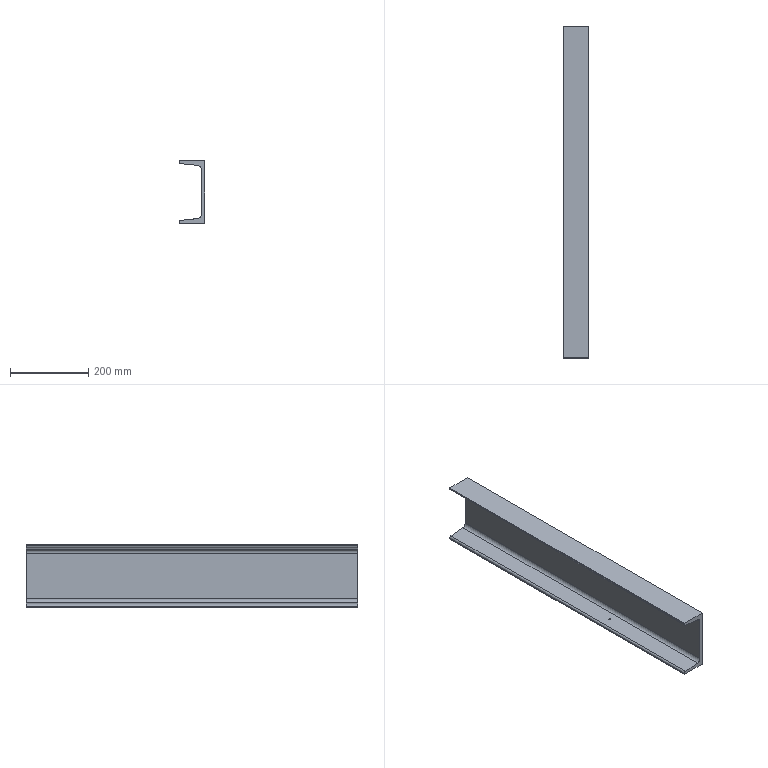Component | SolidWorks | NitrogenSupportChannelSteel65016a-331MachineTool-1 | 1 solid | 16 faces | box 65 x 850 x 160 mm | volume 2137904 mm3 | plane 10 | cylinder 6 | commonest cylinder face diameters 5 x2 20 x2 10 x2
STEP:
#1=COLOUR_RGB('',0.7922,0.8196,0.9333);
#2=FILL_AREA_STYLE_COLOUR('',#1);
#3=FILL_AREA_STYLE('',(#2));
#4=SURFACE_STYLE_FILL_AREA(#3);
#5=SURFACE_SIDE_STYLE('',(#4));
#6=SURFACE_STYLE_USAGE(.BOTH.,#5);
#7=PRESENTATION_STYLE_ASSIGNMENT((#6));
#8=CARTESIAN_POINT('',(1.747,6.759,23.228));
#9=VERTEX_POINT('',#8);
#10=CARTESIAN_POINT('',(1.945,6.759,23.228));
#11=VERTEX_POINT('',#10);
#12=CARTESIAN_POINT('',(1.747,6.759,23.228));
#13=CARTESIAN_POINT('',(1.747,6.956,23.228));
#14=CARTESIAN_POINT('',(1.945,6.956,23.228));
#15=CARTESIAN_POINT('',(1.945,6.759,23.228));
#16=(BOUNDED_CURVE()B_SPLINE_CURVE(3,(#12,#13,#14,#15),.UNSPECIFIED.,.F.,.T.)B_SPLINE_CURVE_WITH_KNOTS((4,4),(0.,3.142),.UNSPECIFIED.)CURVE()GEOMETRIC_REPRESENTATION_ITEM()RATIONAL_B_SPLINE_CURVE((1.,0.3333,0.3333,1.))REPRESENTATION_ITEM(''));
#17=EDGE_CURVE('',#9,#11,#16,.T.);
#18=ORIENTED_EDGE('',*,*,#17,.T.);
#19=CARTESIAN_POINT('',(1.905,6.759,23.632));
#20=VERTEX_POINT('',#19);
#21=CARTESIAN_POINT('',(1.905,6.759,23.632));
#22=DIRECTION('',(-0.0995,0.,0.995));
#23=VECTOR('',#22,39.37);
#24=LINE('',#21,#23);
#25=EDGE_CURVE('',#11,#20,#24,.T.);
#26=ORIENTED_EDGE('',*,*,#25,.T.);
#27=CARTESIAN_POINT('',(1.709,6.759,23.612));
#28=VERTEX_POINT('',#27);
#29=CARTESIAN_POINT('',(1.807,6.759,23.622));
#30=DIRECTION('',(-0.0995,0.,0.995));
#31=DIRECTION('',(-0.995,0.,-0.0995));
#32=AXIS2_PLACEMENT_3D('',#29,#30,#31);
#33=CIRCLE('',#32,0.09843);
#34=EDGE_CURVE('',#20,#28,#33,.T.);
#35=ORIENTED_EDGE('',*,*,#34,.T.);
#36=CARTESIAN_POINT('',(1.709,6.759,23.612));
#37=DIRECTION('',(-0.0995,0.,0.995));
#38=VECTOR('',#37,39.37);
#39=LINE('',#36,#38);
#40=EDGE_CURVE('',#9,#28,#39,.T.);
#41=ORIENTED_EDGE('',*,*,#40,.F.);
#42=EDGE_LOOP('',(#18,#26,#35,#41));
#43=FACE_OUTER_BOUND('',#42,.T.);
#44=CARTESIAN_POINT('',(1.807,6.759,23.622));
#45=DIRECTION('',(-0.0995,0.,0.995));
#46=DIRECTION('',(-0.995,0.,-0.0995));
#47=AXIS2_PLACEMENT_3D('',#44,#45,#46);
#48=CYLINDRICAL_SURFACE('',#47,0.09843);
#49=ADVANCED_FACE('',(#43),#48,.F.);
#50=CARTESIAN_POINT('',(2.567,28.482,23.698));
#51=VERTEX_POINT('',#50);
#52=CARTESIAN_POINT('',(2.922,28.482,24.09));
#53=VERTEX_POINT('',#52);
#54=CARTESIAN_POINT('',(2.528,28.482,24.09));
#55=DIRECTION('',(0.,-1.,-0.));
#56=DIRECTION('',(-1.,0.,0.));
#57=AXIS2_PLACEMENT_3D('',#54,#55,#56);
#58=CIRCLE('',#57,0.3937);
#59=EDGE_CURVE('',#51,#53,#58,.T.);
#60=ORIENTED_EDGE('',*,*,#59,.F.);
#61=CARTESIAN_POINT('',(2.567,-4.983,23.698));
#62=VERTEX_POINT('',#61);
#63=CARTESIAN_POINT('',(2.567,-4.983,23.698));
#64=DIRECTION('',(-0.,1.,0.));
#65=VECTOR('',#64,39.37);
#66=LINE('',#63,#65);
#67=EDGE_CURVE('',#62,#51,#66,.T.);
#68=ORIENTED_EDGE('',*,*,#67,.F.);
#69=CARTESIAN_POINT('',(2.922,-4.983,24.09));
#70=VERTEX_POINT('',#69);
#71=CARTESIAN_POINT('',(2.528,-4.983,24.09));
#72=DIRECTION('',(0.,-1.,-0.));
#73=DIRECTION('',(-1.,0.,0.));
#74=AXIS2_PLACEMENT_3D('',#71,#72,#73);
#75=CIRCLE('',#74,0.3937);
#76=EDGE_CURVE('',#62,#70,#75,.T.);
#77=ORIENTED_EDGE('',*,*,#76,.T.);
#78=CARTESIAN_POINT('',(2.922,-4.983,24.09));
#79=DIRECTION('',(-0.,1.,0.));
#80=VECTOR('',#79,39.37);
#81=LINE('',#78,#80);
#82=EDGE_CURVE('',#70,#53,#81,.T.);
#83=ORIENTED_EDGE('',*,*,#82,.T.);
#84=EDGE_LOOP('',(#60,#68,#77,#83));
#85=FACE_OUTER_BOUND('',#84,.T.);
#86=CARTESIAN_POINT('',(2.528,-4.983,24.09));
#87=DIRECTION('',(-0.,1.,0.));
#88=DIRECTION('',(1.,0.,0.));
#89=AXIS2_PLACEMENT_3D('',#86,#87,#88);
#90=CYLINDRICAL_SURFACE('',#89,0.3937);
#91=ADVANCED_FACE('',(#85),#90,.F.);
#92=CARTESIAN_POINT('',(1.807,6.759,23.622));
#93=DIRECTION('',(-0.0995,0.,0.995));
#94=DIRECTION('',(-0.995,0.,-0.0995));
#95=AXIS2_PLACEMENT_3D('',#92,#93,#94);
#96=CIRCLE('',#95,0.09843);
#97=EDGE_CURVE('',#28,#20,#96,.T.);
#98=ORIENTED_EDGE('',*,*,#97,.F.);
#99=ORIENTED_EDGE('',*,*,#34,.F.);
#100=EDGE_LOOP('',(#98,#99));
#101=FACE_BOUND('',#100,.T.);
#102=CARTESIAN_POINT('',(0.8749,28.482,23.529));
#103=VERTEX_POINT('',#102);
#104=CARTESIAN_POINT('',(0.8749,28.482,23.529));
#105=DIRECTION('',(0.995,-0.,0.0995));
#106=VECTOR('',#105,39.37);
#107=LINE('',#104,#106);
#108=EDGE_CURVE('',#103,#51,#107,.T.);
#109=ORIENTED_EDGE('',*,*,#108,.F.);
#110=CARTESIAN_POINT('',(0.8749,-4.983,23.529));
#111=VERTEX_POINT('',#110);
#112=CARTESIAN_POINT('',(0.8749,-4.983,23.529));
#113=DIRECTION('',(-0.,1.,0.));
#114=VECTOR('',#113,39.37);
#115=LINE('',#112,#114);
#116=EDGE_CURVE('',#111,#103,#115,.T.);
#117=ORIENTED_EDGE('',*,*,#116,.F.);
#118=CARTESIAN_POINT('',(0.8749,-4.983,23.529));
#119=DIRECTION('',(0.995,-0.,0.0995));
#120=VECTOR('',#119,39.37);
#121=LINE('',#118,#120);
#122=EDGE_CURVE('',#111,#62,#121,.T.);
#123=ORIENTED_EDGE('',*,*,#122,.T.);
#124=ORIENTED_EDGE('',*,*,#67,.T.);
#125=EDGE_LOOP('',(#109,#117,#123,#124));
#126=FACE_OUTER_BOUND('',#125,.T.);
#127=CARTESIAN_POINT('',(0.8749,-4.983,23.529));
#128=DIRECTION('',(-0.0995,0.,0.995));
#129=DIRECTION('',(-0.995,0.,-0.0995));
#130=AXIS2_PLACEMENT_3D('',#127,#128,#129);
#131=PLANE('',#130);
#132=ADVANCED_FACE('',(#101,#126),#131,.T.);
#133=CARTESIAN_POINT('',(0.6976,28.482,23.333));
#134=VERTEX_POINT('',#133);
#135=CARTESIAN_POINT('',(0.8945,28.482,23.333));
#136=DIRECTION('',(-0.,1.,0.));
#137=DIRECTION('',(1.,0.,0.));
#138=AXIS2_PLACEMENT_3D('',#135,#136,#137);
#139=CIRCLE('',#138,0.1969);
#140=EDGE_CURVE('',#134,#103,#139,.T.);
#141=ORIENTED_EDGE('',*,*,#140,.F.);
#142=CARTESIAN_POINT('',(0.6976,-4.983,23.333));
#143=VERTEX_POINT('',#142);
#144=CARTESIAN_POINT('',(0.6976,-4.983,23.333));
#145=DIRECTION('',(-0.,1.,0.));
#146=VECTOR('',#145,39.37);
#147=LINE('',#144,#146);
#148=EDGE_CURVE('',#143,#134,#147,.T.);
#149=ORIENTED_EDGE('',*,*,#148,.F.);
#150=CARTESIAN_POINT('',(0.8945,-4.983,23.333));
#151=DIRECTION('',(-0.,1.,0.));
#152=DIRECTION('',(1.,0.,0.));
#153=AXIS2_PLACEMENT_3D('',#150,#151,#152);
#154=CIRCLE('',#153,0.1969);
#155=EDGE_CURVE('',#143,#111,#154,.T.);
#156=ORIENTED_EDGE('',*,*,#155,.T.);
#157=ORIENTED_EDGE('',*,*,#116,.T.);
#158=EDGE_LOOP('',(#141,#149,#156,#157));
#159=FACE_OUTER_BOUND('',#158,.T.);
#160=CARTESIAN_POINT('',(0.8945,-4.983,23.333));
#161=DIRECTION('',(-0.,1.,0.));
#162=DIRECTION('',(1.,0.,0.));
#163=AXIS2_PLACEMENT_3D('',#160,#161,#162);
#164=CYLINDRICAL_SURFACE('',#163,0.1969);
#165=ADVANCED_FACE('',(#159),#164,.T.);
#166=CARTESIAN_POINT('',(0.6976,28.482,23.228));
#167=VERTEX_POINT('',#166);
#168=CARTESIAN_POINT('',(0.6976,28.482,23.228));
#169=DIRECTION('',(-0.,0.,1.));
#170=VECTOR('',#169,39.37);
#171=LINE('',#168,#170);
#172=EDGE_CURVE('',#167,#134,#171,.T.);
#173=ORIENTED_EDGE('',*,*,#172,.F.);
#174=CARTESIAN_POINT('',(0.6976,-4.983,23.228));
#175=VERTEX_POINT('',#174);
#176=CARTESIAN_POINT('',(0.6976,-4.983,23.228));
#177=DIRECTION('',(-0.,1.,0.));
#178=VECTOR('',#177,39.37);
#179=LINE('',#176,#178);
#180=EDGE_CURVE('',#175,#167,#179,.T.);
#181=ORIENTED_EDGE('',*,*,#180,.F.);
#182=CARTESIAN_POINT('',(0.6976,-4.983,23.228));
#183=DIRECTION('',(-0.,0.,1.));
#184=VECTOR('',#183,39.37);
#185=LINE('',#182,#184);
#186=EDGE_CURVE('',#175,#143,#185,.T.);
#187=ORIENTED_EDGE('',*,*,#186,.T.);
#188=ORIENTED_EDGE('',*,*,#148,.T.);
#189=EDGE_LOOP('',(#173,#181,#187,#188));
#190=FACE_OUTER_BOUND('',#189,.T.);
#191=CARTESIAN_POINT('',(0.6976,-4.983,23.228));
#192=DIRECTION('',(-1.,-0.,0.));
#193=DIRECTION('',(-0.,1.,0.));
#194=AXIS2_PLACEMENT_3D('',#191,#192,#193);
#195=PLANE('',#194);
#196=ADVANCED_FACE('',(#190),#195,.T.);
#197=ORIENTED_EDGE('',*,*,#17,.F.);
#198=CARTESIAN_POINT('',(1.945,6.759,23.228));
#199=CARTESIAN_POINT('',(1.945,6.563,23.228));
#200=CARTESIAN_POINT('',(1.747,6.563,23.228));
#201=CARTESIAN_POINT('',(1.747,6.759,23.228));
#202=(BOUNDED_CURVE()B_SPLINE_CURVE(3,(#198,#199,#200,#201),.UNSPECIFIED.,.F.,.T.)B_SPLINE_CURVE_WITH_KNOTS((4,4),(3.142,6.283),.UNSPECIFIED.)CURVE()GEOMETRIC_REPRESENTATION_ITEM()RATIONAL_B_SPLINE_CURVE((1.,0.3333,0.3333,1.))REPRESENTATION_ITEM(''));
#203=EDGE_CURVE('',#11,#9,#202,.T.);
#204=ORIENTED_EDGE('',*,*,#203,.F.);
#205=EDGE_LOOP('',(#197,#204));
#206=FACE_BOUND('',#205,.T.);
#207=CARTESIAN_POINT('',(3.257,28.482,23.228));
#208=VERTEX_POINT('',#207);
#209=CARTESIAN_POINT('',(3.257,28.482,23.228));
#210=DIRECTION('',(-1.,0.,0.));
#211=VECTOR('',#210,39.37);
#212=LINE('',#209,#211);
#213=EDGE_CURVE('',#208,#167,#212,.T.);
#214=ORIENTED_EDGE('',*,*,#213,.F.);
#215=CARTESIAN_POINT('',(3.257,-4.983,23.228));
#216=VERTEX_POINT('',#215);
#217=CARTESIAN_POINT('',(3.257,-4.983,23.228));
#218=DIRECTION('',(-0.,1.,0.));
#219=VECTOR('',#218,39.37);
#220=LINE('',#217,#219);
#221=EDGE_CURVE('',#216,#208,#220,.T.);
#222=ORIENTED_EDGE('',*,*,#221,.F.);
#223=CARTESIAN_POINT('',(3.257,-4.983,23.228));
#224=DIRECTION('',(-1.,0.,0.));
#225=VECTOR('',#224,39.37);
#226=LINE('',#223,#225);
#227=EDGE_CURVE('',#216,#175,#226,.T.);
#228=ORIENTED_EDGE('',*,*,#227,.T.);
#229=ORIENTED_EDGE('',*,*,#180,.T.);
#230=EDGE_LOOP('',(#214,#222,#228,#229));
#231=FACE_OUTER_BOUND('',#230,.T.);
#232=CARTESIAN_POINT('',(3.257,-4.983,23.228));
#233=DIRECTION('',(0.,0.,-1.));
#234=DIRECTION('',(0.,-1.,-0.));
#235=AXIS2_PLACEMENT_3D('',#232,#233,#234);
#236=PLANE('',#235);
#237=ADVANCED_FACE('',(#206,#231),#236,.T.);
#238=CARTESIAN_POINT('',(3.257,28.482,29.528));
#239=VERTEX_POINT('',#238);
#240=CARTESIAN_POINT('',(3.257,28.482,29.528));
#241=DIRECTION('',(0.,-0.,-1.));
#242=VECTOR('',#241,39.37);
#243=LINE('',#240,#242);
#244=EDGE_CURVE('',#239,#208,#243,.T.);
#245=ORIENTED_EDGE('',*,*,#244,.F.);
#246=CARTESIAN_POINT('',(3.257,-4.983,29.528));
#247=VERTEX_POINT('',#246);
#248=CARTESIAN_POINT('',(3.257,-4.983,29.528));
#249=DIRECTION('',(-0.,1.,0.));
#250=VECTOR('',#249,39.37);
#251=LINE('',#248,#250);
#252=EDGE_CURVE('',#247,#239,#251,.T.);
#253=ORIENTED_EDGE('',*,*,#252,.F.);
#254=CARTESIAN_POINT('',(3.257,-4.983,29.528));
#255=DIRECTION('',(0.,-0.,-1.));
#256=VECTOR('',#255,39.37);
#257=LINE('',#254,#256);
#258=EDGE_CURVE('',#247,#216,#257,.T.);
#259=ORIENTED_EDGE('',*,*,#258,.T.);
#260=ORIENTED_EDGE('',*,*,#221,.T.);
#261=EDGE_LOOP('',(#245,#253,#259,#260));
#262=FACE_OUTER_BOUND('',#261,.T.);
#263=CARTESIAN_POINT('',(3.257,-4.983,29.528));
#264=DIRECTION('',(1.,0.,-0.));
#265=DIRECTION('',(0.,-1.,-0.));
#266=AXIS2_PLACEMENT_3D('',#263,#264,#265);
#267=PLANE('',#266);
#268=ADVANCED_FACE('',(#262),#267,.T.);
#269=CARTESIAN_POINT('',(0.6976,28.482,29.528));
#270=VERTEX_POINT('',#269);
#271=CARTESIAN_POINT('',(0.6976,28.482,29.528));
#272=DIRECTION('',(1.,-0.,-0.));
#273=VECTOR('',#272,39.37);
#274=LINE('',#271,#273);
#275=EDGE_CURVE('',#270,#239,#274,.T.);
#276=ORIENTED_EDGE('',*,*,#275,.F.);
#277=CARTESIAN_POINT('',(0.6976,-4.983,29.528));
#278=VERTEX_POINT('',#277);
#279=CARTESIAN_POINT('',(0.6976,-4.983,29.528));
#280=DIRECTION('',(-0.,1.,0.));
#281=VECTOR('',#280,39.37);
#282=LINE('',#279,#281);
#283=EDGE_CURVE('',#278,#270,#282,.T.);
#284=ORIENTED_EDGE('',*,*,#283,.F.);
#285=CARTESIAN_POINT('',(0.6976,-4.983,29.528));
#286=DIRECTION('',(1.,-0.,-0.));
#287=VECTOR('',#286,39.37);
#288=LINE('',#285,#287);
#289=EDGE_CURVE('',#278,#247,#288,.T.);
#290=ORIENTED_EDGE('',*,*,#289,.T.);
#291=ORIENTED_EDGE('',*,*,#252,.T.);
#292=EDGE_LOOP('',(#276,#284,#290,#291));
#293=FACE_OUTER_BOUND('',#292,.T.);
#294=CARTESIAN_POINT('',(0.6976,-4.983,29.528));
#295=DIRECTION('',(-0.,-0.,1.));
#296=DIRECTION('',(-0.,1.,0.));
#297=AXIS2_PLACEMENT_3D('',#294,#295,#296);
#298=PLANE('',#297);
#299=ADVANCED_FACE('',(#293),#298,.T.);
#300=CARTESIAN_POINT('',(0.6976,28.482,29.423));
#301=VERTEX_POINT('',#300);
#302=CARTESIAN_POINT('',(0.6976,28.482,29.423));
#303=DIRECTION('',(-0.,0.,1.));
#304=VECTOR('',#303,39.37);
#305=LINE('',#302,#304);
#306=EDGE_CURVE('',#301,#270,#305,.T.);
#307=ORIENTED_EDGE('',*,*,#306,.F.);
#308=CARTESIAN_POINT('',(0.6976,-4.983,29.423));
#309=VERTEX_POINT('',#308);
#310=CARTESIAN_POINT('',(0.6976,-4.983,29.423));
#311=DIRECTION('',(-0.,1.,0.));
#312=VECTOR('',#311,39.37);
#313=LINE('',#310,#312);
#314=EDGE_CURVE('',#309,#301,#313,.T.);
#315=ORIENTED_EDGE('',*,*,#314,.F.);
#316=CARTESIAN_POINT('',(0.6976,-4.983,29.423));
#317=DIRECTION('',(-0.,0.,1.));
#318=VECTOR('',#317,39.37);
#319=LINE('',#316,#318);
#320=EDGE_CURVE('',#309,#278,#319,.T.);
#321=ORIENTED_EDGE('',*,*,#320,.T.);
#322=ORIENTED_EDGE('',*,*,#283,.T.);
#323=EDGE_LOOP('',(#307,#315,#321,#322));
#324=FACE_OUTER_BOUND('',#323,.T.);
#325=CARTESIAN_POINT('',(0.6976,-4.983,29.423));
#326=DIRECTION('',(-1.,-0.,0.));
#327=DIRECTION('',(-0.,1.,0.));
#328=AXIS2_PLACEMENT_3D('',#325,#326,#327);
#329=PLANE('',#328);
#330=ADVANCED_FACE('',(#324),#329,.T.);
#331=CARTESIAN_POINT('',(0.8749,28.482,29.227));
#332=VERTEX_POINT('',#331);
#333=CARTESIAN_POINT('',(0.8945,28.482,29.423));
#334=DIRECTION('',(-0.,1.,0.));
#335=DIRECTION('',(1.,0.,0.));
#336=AXIS2_PLACEMENT_3D('',#333,#334,#335);
#337=CIRCLE('',#336,0.1969);
#338=EDGE_CURVE('',#332,#301,#337,.T.);
#339=ORIENTED_EDGE('',*,*,#338,.F.);
#340=CARTESIAN_POINT('',(0.8749,-4.983,29.227));
#341=VERTEX_POINT('',#340);
#342=CARTESIAN_POINT('',(0.8749,-4.983,29.227));
#343=DIRECTION('',(-0.,1.,0.));
#344=VECTOR('',#343,39.37);
#345=LINE('',#342,#344);
#346=EDGE_CURVE('',#341,#332,#345,.T.);
#347=ORIENTED_EDGE('',*,*,#346,.F.);
#348=CARTESIAN_POINT('',(0.8945,-4.983,29.423));
#349=DIRECTION('',(-0.,1.,0.));
#350=DIRECTION('',(1.,0.,0.));
#351=AXIS2_PLACEMENT_3D('',#348,#349,#350);
#352=CIRCLE('',#351,0.1969);
#353=EDGE_CURVE('',#341,#309,#352,.T.);
#354=ORIENTED_EDGE('',*,*,#353,.T.);
#355=ORIENTED_EDGE('',*,*,#314,.T.);
#356=EDGE_LOOP('',(#339,#347,#354,#355));
#357=FACE_OUTER_BOUND('',#356,.T.);
#358=CARTESIAN_POINT('',(0.8945,-4.983,29.423));
#359=DIRECTION('',(-0.,1.,0.));
#360=DIRECTION('',(1.,0.,0.));
#361=AXIS2_PLACEMENT_3D('',#358,#359,#360);
#362=CYLINDRICAL_SURFACE('',#361,0.1969);
#363=ADVANCED_FACE('',(#357),#362,.T.);
#364=CARTESIAN_POINT('',(2.567,28.482,29.058));
#365=VERTEX_POINT('',#364);
#366=CARTESIAN_POINT('',(2.567,28.482,29.058));
#367=DIRECTION('',(-0.995,0.,0.0995));
#368=VECTOR('',#367,39.37);
#369=LINE('',#366,#368);
#370=EDGE_CURVE('',#365,#332,#369,.T.);
#371=ORIENTED_EDGE('',*,*,#370,.F.);
#372=CARTESIAN_POINT('',(2.567,-4.983,29.058));
#373=VERTEX_POINT('',#372);
#374=CARTESIAN_POINT('',(2.567,-4.983,29.058));
#375=DIRECTION('',(-0.,1.,0.));
#376=VECTOR('',#375,39.37);
#377=LINE('',#374,#376);
#378=EDGE_CURVE('',#373,#365,#377,.T.);
#379=ORIENTED_EDGE('',*,*,#378,.F.);
#380=CARTESIAN_POINT('',(2.567,-4.983,29.058));
#381=DIRECTION('',(-0.995,0.,0.0995));
#382=VECTOR('',#381,39.37);
#383=LINE('',#380,#382);
#384=EDGE_CURVE('',#373,#341,#383,.T.);
#385=ORIENTED_EDGE('',*,*,#384,.T.);
#386=ORIENTED_EDGE('',*,*,#346,.T.);
#387=EDGE_LOOP('',(#371,#379,#385,#386));
#388=FACE_OUTER_BOUND('',#387,.T.);
#389=CARTESIAN_POINT('',(2.567,-4.983,29.058));
#390=DIRECTION('',(-0.0995,0.,-0.995));
#391=DIRECTION('',(0.995,-0.,-0.0995));
#392=AXIS2_PLACEMENT_3D('',#389,#390,#391);
#393=PLANE('',#392);
#394=ADVANCED_FACE('',(#388),#393,.T.);
#395=CARTESIAN_POINT('',(2.922,28.482,28.666));
#396=VERTEX_POINT('',#395);
#397=CARTESIAN_POINT('',(2.528,28.482,28.666));
#398=DIRECTION('',(0.,-1.,-0.));
#399=DIRECTION('',(-1.,0.,0.));
#400=AXIS2_PLACEMENT_3D('',#397,#398,#399);
#401=CIRCLE('',#400,0.3937);
#402=EDGE_CURVE('',#396,#365,#401,.T.);
#403=ORIENTED_EDGE('',*,*,#402,.F.);
#404=CARTESIAN_POINT('',(2.922,-4.983,28.666));
#405=VERTEX_POINT('',#404);
#406=CARTESIAN_POINT('',(2.922,-4.983,28.666));
#407=DIRECTION('',(-0.,1.,0.));
#408=VECTOR('',#407,39.37);
#409=LINE('',#406,#408);
#410=EDGE_CURVE('',#405,#396,#409,.T.);
#411=ORIENTED_EDGE('',*,*,#410,.F.);
#412=CARTESIAN_POINT('',(2.528,-4.983,28.666));
#413=DIRECTION('',(0.,-1.,-0.));
#414=DIRECTION('',(-1.,0.,0.));
#415=AXIS2_PLACEMENT_3D('',#412,#413,#414);
#416=CIRCLE('',#415,0.3937);
#417=EDGE_CURVE('',#405,#373,#416,.T.);
#418=ORIENTED_EDGE('',*,*,#417,.T.);
#419=ORIENTED_EDGE('',*,*,#378,.T.);
#420=EDGE_LOOP('',(#403,#411,#418,#419));
#421=FACE_OUTER_BOUND('',#420,.T.);
#422=CARTESIAN_POINT('',(2.528,-4.983,28.666));
#423=DIRECTION('',(-0.,1.,0.));
#424=DIRECTION('',(1.,0.,0.));
#425=AXIS2_PLACEMENT_3D('',#422,#423,#424);
#426=CYLINDRICAL_SURFACE('',#425,0.3937);
#427=ADVANCED_FACE('',(#421),#426,.F.);
#428=CARTESIAN_POINT('',(2.922,28.482,24.09));
#429=DIRECTION('',(0.,0.,1.));
#430=VECTOR('',#429,39.37);
#431=LINE('',#428,#430);
#432=EDGE_CURVE('',#53,#396,#431,.T.);
#433=ORIENTED_EDGE('',*,*,#432,.F.);
#434=ORIENTED_EDGE('',*,*,#82,.F.);
#435=CARTESIAN_POINT('',(2.922,-4.983,24.09));
#436=DIRECTION('',(0.,0.,1.));
#437=VECTOR('',#436,39.37);
#438=LINE('',#435,#437);
#439=EDGE_CURVE('',#70,#405,#438,.T.);
#440=ORIENTED_EDGE('',*,*,#439,.T.);
#441=ORIENTED_EDGE('',*,*,#410,.T.);
#442=EDGE_LOOP('',(#433,#434,#440,#441));
#443=FACE_OUTER_BOUND('',#442,.T.);
#444=CARTESIAN_POINT('',(2.922,-4.983,24.09));
#445=DIRECTION('',(-1.,0.,0.));
#446=DIRECTION('',(-0.,-0.,-1.));
#447=AXIS2_PLACEMENT_3D('',#444,#445,#446);
#448=PLANE('',#447);
#449=ADVANCED_FACE('',(#443),#448,.T.);
#450=ORIENTED_EDGE('',*,*,#76,.F.);
#451=ORIENTED_EDGE('',*,*,#122,.F.);
#452=ORIENTED_EDGE('',*,*,#155,.F.);
#453=ORIENTED_EDGE('',*,*,#186,.F.);
#454=ORIENTED_EDGE('',*,*,#227,.F.);
#455=ORIENTED_EDGE('',*,*,#258,.F.);
#456=ORIENTED_EDGE('',*,*,#289,.F.);
#457=ORIENTED_EDGE('',*,*,#320,.F.);
#458=ORIENTED_EDGE('',*,*,#353,.F.);
#459=ORIENTED_EDGE('',*,*,#384,.F.);
#460=ORIENTED_EDGE('',*,*,#417,.F.);
#461=ORIENTED_EDGE('',*,*,#439,.F.);
#462=EDGE_LOOP('',(#450,#451,#452,#453,#454,#455,#456,#457,#458,#459,#460,#461));
#463=FACE_OUTER_BOUND('',#462,.T.);
#464=CARTESIAN_POINT('',(2.528,-4.983,24.09));
#465=DIRECTION('',(-0.,-1.,-0.));
#466=DIRECTION('',(-1.,0.,0.));
#467=AXIS2_PLACEMENT_3D('',#464,#465,#466);
#468=PLANE('',#467);
#469=ADVANCED_FACE('',(#463),#468,.T.);
#470=ORIENTED_EDGE('',*,*,#59,.T.);
#471=ORIENTED_EDGE('',*,*,#432,.T.);
#472=ORIENTED_EDGE('',*,*,#402,.T.);
#473=ORIENTED_EDGE('',*,*,#370,.T.);
#474=ORIENTED_EDGE('',*,*,#338,.T.);
#475=ORIENTED_EDGE('',*,*,#306,.T.);
#476=ORIENTED_EDGE('',*,*,#275,.T.);
#477=ORIENTED_EDGE('',*,*,#244,.T.);
#478=ORIENTED_EDGE('',*,*,#213,.T.);
#479=ORIENTED_EDGE('',*,*,#172,.T.);
#480=ORIENTED_EDGE('',*,*,#140,.T.);
#481=ORIENTED_EDGE('',*,*,#108,.T.);
#482=EDGE_LOOP('',(#470,#471,#472,#473,#474,#475,#476,#477,#478,#479,#480,#481));
#483=FACE_OUTER_BOUND('',#482,.T.);
#484=CARTESIAN_POINT('',(2.528,28.482,24.09));
#485=DIRECTION('',(-0.,-1.,-0.));
#486=DIRECTION('',(-1.,0.,0.));
#487=AXIS2_PLACEMENT_3D('',#484,#485,#486);
#488=PLANE('',#487);
#489=ADVANCED_FACE('',(#483),#488,.F.);
#490=ORIENTED_EDGE('',*,*,#25,.F.);
#491=ORIENTED_EDGE('',*,*,#203,.T.);
#492=ORIENTED_EDGE('',*,*,#40,.T.);
#493=ORIENTED_EDGE('',*,*,#97,.T.);
#494=EDGE_LOOP('',(#490,#491,#492,#493));
#495=FACE_OUTER_BOUND('',#494,.T.);
#496=CARTESIAN_POINT('',(1.807,6.759,23.622));
#497=DIRECTION('',(-0.0995,0.,0.995));
#498=DIRECTION('',(-0.995,0.,-0.0995));
#499=AXIS2_PLACEMENT_3D('',#496,#497,#498);
#500=CYLINDRICAL_SURFACE('',#499,0.09843);
#501=ADVANCED_FACE('',(#495),#500,.F.);
#502=CLOSED_SHELL('',(#49,#91,#132,#165,#196,#237,#268,#299,#330,#363,#394,#427,#449,#469,#489,#501));
#503=MANIFOLD_SOLID_BREP('',#502);
#504=STYLED_ITEM('',(#7),#503);
#505=PRESENTATION_LAYER_ASSIGNMENT('','',(#504));
#506=CARTESIAN_POINT('',(0.,0.,0.));
#507=DIRECTION('',(0.,0.,1.));
#508=DIRECTION('',(1.,0.,0.));
#509=AXIS2_PLACEMENT_3D('',#506,#507,#508);
#510=(LENGTH_UNIT()NAMED_UNIT(*)SI_UNIT($,.METRE.));
#511=LENGTH_MEASURE_WITH_UNIT(LENGTH_MEASURE(0.0254),#510);
#512=DIMENSIONAL_EXPONENTS(1.,0.,0.,0.,0.,0.,0.);
#513=(CONVERSION_BASED_UNIT('',#511)LENGTH_UNIT()NAMED_UNIT(#512));
#514=UNCERTAINTY_MEASURE_WITH_UNIT(LENGTH_MEASURE(0.00001),#513,'','');
#515=(NAMED_UNIT(*)PLANE_ANGLE_UNIT()SI_UNIT($,.RADIAN.));
#516=(NAMED_UNIT(*)SI_UNIT($,.STERADIAN.)SOLID_ANGLE_UNIT());
#517=(GEOMETRIC_REPRESENTATION_CONTEXT(3)GLOBAL_UNCERTAINTY_ASSIGNED_CONTEXT((#514))GLOBAL_UNIT_ASSIGNED_CONTEXT((#513,#515,#516))REPRESENTATION_CONTEXT('',''));
#518=ADVANCED_BREP_SHAPE_REPRESENTATION('',(#503,#509),#517);
#519=(LENGTH_UNIT()NAMED_UNIT(*)SI_UNIT($,.METRE.));
#520=LENGTH_MEASURE_WITH_UNIT(LENGTH_MEASURE(0.0254),#519);
#521=DIMENSIONAL_EXPONENTS(1.,0.,0.,0.,0.,0.,0.);
#522=(CONVERSION_BASED_UNIT('',#520)LENGTH_UNIT()NAMED_UNIT(#521));
#523=UNCERTAINTY_MEASURE_WITH_UNIT(LENGTH_MEASURE(0.00001),#522,'','');
#524=(NAMED_UNIT(*)PLANE_ANGLE_UNIT()SI_UNIT($,.RADIAN.));
#525=(NAMED_UNIT(*)SI_UNIT($,.STERADIAN.)SOLID_ANGLE_UNIT());
#526=(GEOMETRIC_REPRESENTATION_CONTEXT(3)GLOBAL_UNCERTAINTY_ASSIGNED_CONTEXT((#523))GLOBAL_UNIT_ASSIGNED_CONTEXT((#522,#524,#525))REPRESENTATION_CONTEXT('',''));
#527=MECHANICAL_DESIGN_GEOMETRIC_PRESENTATION_REPRESENTATION('',(#504),#526);